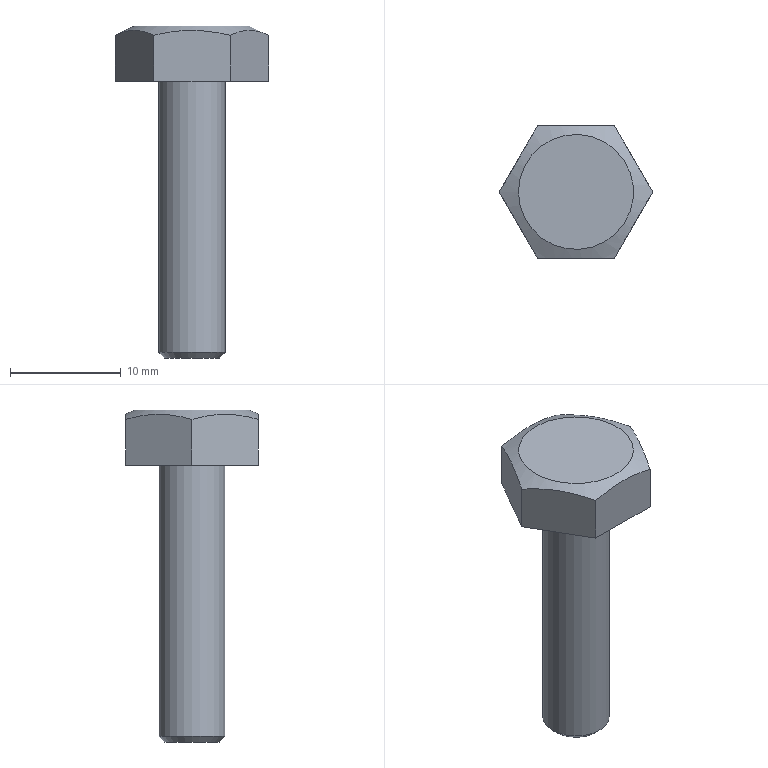Component | NX | BOLT_M6X25 | 1 solid | 12 faces | box 13.86 x 12 x 30 mm | volume 1316 mm3 | plane 9 | cone 2 | cylinder 1 | commonest cylinder face diameters 6 x1
STEP:
#1=CARTESIAN_POINT('',(0.,0.,0.));
#2=DIRECTION('',(0.,0.,1.));
#3=DIRECTION('',(1.,0.,0.));
#4=AXIS2_PLACEMENT_3D('',#1,#2,#3);
#5=CARTESIAN_POINT('',(16.5,-20.,-3.));
#6=VERTEX_POINT('',#5);
#7=CARTESIAN_POINT('',(19.,-20.,-3.));
#8=DIRECTION('',(0.,0.,-1.));
#9=DIRECTION('',(-1.,0.,0.));
#10=AXIS2_PLACEMENT_3D('',#7,#8,#9);
#11=CIRCLE('',#10,2.5);
#12=CARTESIAN_POINT('',(19.,-20.,-3.));
#13=DIRECTION('',(0.,0.,-1.));
#14=DIRECTION('',(-1.,0.,0.));
#15=AXIS2_PLACEMENT_3D('',#12,#13,#14);
#16=PLANE('',#15);
#17=CARTESIAN_POINT('',(0.,0.));
#18=DIRECTION('',(1.,0.));
#19=AXIS2_PLACEMENT_2D('',#17,#18);
#20=CIRCLE('',#19,2.5);
#21=(GEOMETRIC_REPRESENTATION_CONTEXT(2)PARAMETRIC_REPRESENTATION_CONTEXT()REPRESENTATION_CONTEXT('',''));
#22=DEFINITIONAL_REPRESENTATION('',(#20),#21);
#23=PCURVE('',#16,#22);
#24=CARTESIAN_POINT('',(19.,-20.,-2.5));
#25=DIRECTION('',(0.,0.,1.));
#26=DIRECTION('',(1.,0.,0.));
#27=AXIS2_PLACEMENT_3D('',#24,#25,#26);
#28=CONICAL_SURFACE('',#27,3.,0.7854);
#29=CARTESIAN_POINT('',(9.425,-0.5));
#30=DIRECTION('',(-1.,0.));
#31=VECTOR('',#30,1.);
#32=LINE('',#29,#31);
#33=(GEOMETRIC_REPRESENTATION_CONTEXT(2)PARAMETRIC_REPRESENTATION_CONTEXT()REPRESENTATION_CONTEXT('',''));
#34=DEFINITIONAL_REPRESENTATION('',(#32),#33);
#35=PCURVE('',#28,#34);
#36=SURFACE_CURVE('',#11,(#23,#35),.PCURVE_S1.);
#37=EDGE_CURVE('',#6,#6,#36,.T.);
#38=ORIENTED_EDGE('',*,*,#37,.T.);
#39=EDGE_LOOP('',(#38));
#40=FACE_BOUND('',#39,.T.);
#41=ADVANCED_FACE('',(#40),#16,.T.);
#42=CARTESIAN_POINT('',(16.,-20.,-2.5));
#43=VERTEX_POINT('',#42);
#44=CARTESIAN_POINT('',(22.,-20.,-2.5));
#45=VERTEX_POINT('',#44);
#46=CARTESIAN_POINT('',(19.,-20.,-2.5));
#47=DIRECTION('',(0.,0.,1.));
#48=DIRECTION('',(-1.,0.,0.));
#49=AXIS2_PLACEMENT_3D('',#46,#47,#48);
#50=CIRCLE('',#49,3.);
#51=CARTESIAN_POINT('',(19.,-20.,-3.));
#52=DIRECTION('',(0.,0.,1.));
#53=DIRECTION('',(1.,0.,0.));
#54=AXIS2_PLACEMENT_3D('',#51,#52,#53);
#55=CYLINDRICAL_SURFACE('',#54,3.);
#56=CARTESIAN_POINT('',(3.142,0.5));
#57=DIRECTION('',(1.,0.));
#58=VECTOR('',#57,1.);
#59=LINE('',#56,#58);
#60=(GEOMETRIC_REPRESENTATION_CONTEXT(2)PARAMETRIC_REPRESENTATION_CONTEXT()REPRESENTATION_CONTEXT('',''));
#61=DEFINITIONAL_REPRESENTATION('',(#59),#60);
#62=PCURVE('',#55,#61);
#63=CARTESIAN_POINT('',(3.142,0.));
#64=DIRECTION('',(1.,0.));
#65=VECTOR('',#64,1.);
#66=LINE('',#63,#65);
#67=(GEOMETRIC_REPRESENTATION_CONTEXT(2)PARAMETRIC_REPRESENTATION_CONTEXT()REPRESENTATION_CONTEXT('',''));
#68=DEFINITIONAL_REPRESENTATION('',(#66),#67);
#69=PCURVE('',#28,#68);
#70=SURFACE_CURVE('',#50,(#62,#69),.PCURVE_S1.);
#71=EDGE_CURVE('',#43,#45,#70,.T.);
#72=ORIENTED_EDGE('',*,*,#71,.T.);
#73=CARTESIAN_POINT('',(22.,-20.,22.));
#74=VERTEX_POINT('',#73);
#75=CARTESIAN_POINT('',(22.,-20.,-2.5));
#76=CARTESIAN_POINT('',(22.,-20.,22.));
#77=B_SPLINE_CURVE_WITH_KNOTS('',1,(#75,#76),.UNSPECIFIED.,.F.,.F.,(2,2),(0.5,25.),.PIECEWISE_BEZIER_KNOTS.);
#78=CARTESIAN_POINT('',(6.283,0.));
#79=DIRECTION('',(0.,1.));
#80=VECTOR('',#79,1.);
#81=LINE('',#78,#80);
#82=(GEOMETRIC_REPRESENTATION_CONTEXT(2)PARAMETRIC_REPRESENTATION_CONTEXT()REPRESENTATION_CONTEXT('',''));
#83=DEFINITIONAL_REPRESENTATION('',(#81),#82);
#84=PCURVE('',#55,#83);
#85=CARTESIAN_POINT('',(0.,0.));
#86=DIRECTION('',(0.,1.));
#87=VECTOR('',#86,1.);
#88=LINE('',#85,#87);
#89=(GEOMETRIC_REPRESENTATION_CONTEXT(2)PARAMETRIC_REPRESENTATION_CONTEXT()REPRESENTATION_CONTEXT('',''));
#90=DEFINITIONAL_REPRESENTATION('',(#88),#89);
#91=PCURVE('',#55,#90);
#92=SEAM_CURVE('',#77,(#84,#91),.PCURVE_S1.);
#93=EDGE_CURVE('',#45,#74,#92,.T.);
#94=ORIENTED_EDGE('',*,*,#93,.T.);
#95=CARTESIAN_POINT('',(19.,-20.,22.));
#96=DIRECTION('',(0.,0.,-1.));
#97=DIRECTION('',(1.,0.,0.));
#98=AXIS2_PLACEMENT_3D('',#95,#96,#97);
#99=CIRCLE('',#98,3.);
#100=CARTESIAN_POINT('',(6.283,25.));
#101=DIRECTION('',(-1.,0.));
#102=VECTOR('',#101,1.);
#103=LINE('',#100,#102);
#104=(GEOMETRIC_REPRESENTATION_CONTEXT(2)PARAMETRIC_REPRESENTATION_CONTEXT()REPRESENTATION_CONTEXT('',''));
#105=DEFINITIONAL_REPRESENTATION('',(#103),#104);
#106=PCURVE('',#55,#105);
#107=CARTESIAN_POINT('',(19.,-20.,22.));
#108=DIRECTION('',(0.,0.,1.));
#109=DIRECTION('',(1.,0.,0.));
#110=AXIS2_PLACEMENT_3D('',#107,#108,#109);
#111=PLANE('',#110);
#112=CARTESIAN_POINT('',(3.,0.));
#113=CARTESIAN_POINT('',(3.,-5.196));
#114=CARTESIAN_POINT('',(-1.5,-2.598));
#115=CARTESIAN_POINT('',(-6.,-0.));
#116=CARTESIAN_POINT('',(-1.5,2.598));
#117=CARTESIAN_POINT('',(3.,5.196));
#118=CARTESIAN_POINT('',(3.,0.));
#119=(BOUNDED_CURVE()B_SPLINE_CURVE(2,(#112,#113,#114,#115,#116,#117,#118),.UNSPECIFIED.,.T.,.F.)B_SPLINE_CURVE_WITH_KNOTS((1,2,2,2,2,1),(-2.094,0.,2.094,4.189,6.283,8.378),.UNSPECIFIED.)CURVE()GEOMETRIC_REPRESENTATION_ITEM()RATIONAL_B_SPLINE_CURVE((1.,0.5,1.,0.5,1.,0.5,1.))REPRESENTATION_ITEM(''));
#120=(GEOMETRIC_REPRESENTATION_CONTEXT(2)PARAMETRIC_REPRESENTATION_CONTEXT()REPRESENTATION_CONTEXT('',''));
#121=DEFINITIONAL_REPRESENTATION('',(#119),#120);
#122=PCURVE('',#111,#121);
#123=SURFACE_CURVE('',#99,(#106,#122),.PCURVE_S1.);
#124=EDGE_CURVE('',#74,#74,#123,.T.);
#125=ORIENTED_EDGE('',*,*,#124,.T.);
#126=ORIENTED_EDGE('',*,*,#93,.F.);
#127=CARTESIAN_POINT('',(19.,-20.,-2.5));
#128=DIRECTION('',(0.,0.,1.));
#129=DIRECTION('',(-1.,0.,0.));
#130=AXIS2_PLACEMENT_3D('',#127,#128,#129);
#131=CIRCLE('',#130,3.);
#132=CARTESIAN_POINT('',(-3.142,0.5));
#133=DIRECTION('',(1.,0.));
#134=VECTOR('',#133,1.);
#135=LINE('',#132,#134);
#136=(GEOMETRIC_REPRESENTATION_CONTEXT(2)PARAMETRIC_REPRESENTATION_CONTEXT()REPRESENTATION_CONTEXT('',''));
#137=DEFINITIONAL_REPRESENTATION('',(#135),#136);
#138=PCURVE('',#55,#137);
#139=CARTESIAN_POINT('',(3.142,0.));
#140=DIRECTION('',(1.,0.));
#141=VECTOR('',#140,1.);
#142=LINE('',#139,#141);
#143=(GEOMETRIC_REPRESENTATION_CONTEXT(2)PARAMETRIC_REPRESENTATION_CONTEXT()REPRESENTATION_CONTEXT('',''));
#144=DEFINITIONAL_REPRESENTATION('',(#142),#143);
#145=PCURVE('',#28,#144);
#146=SURFACE_CURVE('',#131,(#138,#145),.PCURVE_S1.);
#147=EDGE_CURVE('',#45,#43,#146,.T.);
#148=ORIENTED_EDGE('',*,*,#147,.T.);
#149=EDGE_LOOP('',(#72,#94,#125,#126,#148));
#150=FACE_BOUND('',#149,.T.);
#151=ADVANCED_FACE('',(#150),#55,.T.);
#152=CARTESIAN_POINT('',(15.536,-14.,26.151));
#153=VERTEX_POINT('',#152);
#154=CARTESIAN_POINT('',(15.536,-14.,22.));
#155=VERTEX_POINT('',#154);
#156=CARTESIAN_POINT('',(15.536,-14.,27.));
#157=DIRECTION('',(0.,0.,-1.));
#158=VECTOR('',#157,1.);
#159=LINE('',#156,#158);
#160=CARTESIAN_POINT('',(22.464,-14.,27.));
#161=DIRECTION('',(0.,-1.,0.));
#162=DIRECTION('',(1.,0.,0.));
#163=AXIS2_PLACEMENT_3D('',#160,#161,#162);
#164=PLANE('',#163);
#165=CARTESIAN_POINT('',(-6.928,0.));
#166=DIRECTION('',(0.,-1.));
#167=VECTOR('',#166,1.);
#168=LINE('',#165,#167);
#169=(GEOMETRIC_REPRESENTATION_CONTEXT(2)PARAMETRIC_REPRESENTATION_CONTEXT()REPRESENTATION_CONTEXT('',''));
#170=DEFINITIONAL_REPRESENTATION('',(#168),#169);
#171=PCURVE('',#164,#170);
#172=CARTESIAN_POINT('',(15.536,-14.,27.));
#173=DIRECTION('',(0.866,-0.5,0.));
#174=DIRECTION('',(0.5,0.866,0.));
#175=AXIS2_PLACEMENT_3D('',#172,#173,#174);
#176=PLANE('',#175);
#177=CARTESIAN_POINT('',(0.,0.));
#178=DIRECTION('',(0.,-1.));
#179=VECTOR('',#178,1.);
#180=LINE('',#177,#179);
#181=(GEOMETRIC_REPRESENTATION_CONTEXT(2)PARAMETRIC_REPRESENTATION_CONTEXT()REPRESENTATION_CONTEXT('',''));
#182=DEFINITIONAL_REPRESENTATION('',(#180),#181);
#183=PCURVE('',#176,#182);
#184=SURFACE_CURVE('',#159,(#171,#183),.PCURVE_S1.);
#185=EDGE_CURVE('',#153,#155,#184,.T.);
#186=ORIENTED_EDGE('',*,*,#185,.F.);
#187=CARTESIAN_POINT('',(22.464,-14.,26.151));
#188=VERTEX_POINT('',#187);
#189=CARTESIAN_POINT('',(15.536,-14.,26.151));
#190=CARTESIAN_POINT('',(16.672,-14.,26.43));
#191=CARTESIAN_POINT('',(17.839,-14.,26.606));
#192=CARTESIAN_POINT('',(20.161,-14.,26.606));
#193=CARTESIAN_POINT('',(21.337,-14.,26.427));
#194=CARTESIAN_POINT('',(22.464,-14.,26.151));
#195=B_SPLINE_CURVE_WITH_KNOTS('',3,(#189,#190,#191,#192,#193,#194),.UNSPECIFIED.,.F.,.F.,(4,2,4),(0.,0.5,1.),.UNSPECIFIED.);
#196=CARTESIAN_POINT('',(-6.928,-0.8487));
#197=CARTESIAN_POINT('',(-5.792,-0.5703));
#198=CARTESIAN_POINT('',(-4.625,-0.3939));
#199=CARTESIAN_POINT('',(-2.304,-0.3939));
#200=CARTESIAN_POINT('',(-1.127,-0.5725));
#201=CARTESIAN_POINT('',(0.,-0.8487));
#202=B_SPLINE_CURVE_WITH_KNOTS('',3,(#196,#197,#198,#199,#200,#201),.UNSPECIFIED.,.F.,.F.,(4,2,4),(0.,0.5,1.),.UNSPECIFIED.);
#203=(GEOMETRIC_REPRESENTATION_CONTEXT(2)PARAMETRIC_REPRESENTATION_CONTEXT()REPRESENTATION_CONTEXT('',''));
#204=DEFINITIONAL_REPRESENTATION('',(#202),#203);
#205=PCURVE('',#164,#204);
#206=CARTESIAN_POINT('',(19.,-20.,27.));
#207=DIRECTION('',(0.,0.,-1.));
#208=DIRECTION('',(-1.,0.,0.));
#209=AXIS2_PLACEMENT_3D('',#206,#207,#208);
#210=CONICAL_SURFACE('',#209,5.196,1.115);
#211=CARTESIAN_POINT('',(1.047,0.8487));
#212=CARTESIAN_POINT('',(1.06,0.8234));
#213=CARTESIAN_POINT('',(1.087,0.7744));
#214=CARTESIAN_POINT('',(1.128,0.7061));
#215=CARTESIAN_POINT('',(1.172,0.6434));
#216=CARTESIAN_POINT('',(1.217,0.5869));
#217=CARTESIAN_POINT('',(1.264,0.5368));
#218=CARTESIAN_POINT('',(1.313,0.4937));
#219=CARTESIAN_POINT('',(1.362,0.4578));
#220=CARTESIAN_POINT('',(1.414,0.4295));
#221=CARTESIAN_POINT('',(1.465,0.409));
#222=CARTESIAN_POINT('',(1.518,0.3967));
#223=CARTESIAN_POINT('',(1.571,0.3925));
#224=CARTESIAN_POINT('',(1.624,0.3967));
#225=CARTESIAN_POINT('',(1.676,0.4091));
#226=CARTESIAN_POINT('',(1.728,0.4296));
#227=CARTESIAN_POINT('',(1.779,0.458));
#228=CARTESIAN_POINT('',(1.829,0.4941));
#229=CARTESIAN_POINT('',(1.878,0.5374));
#230=CARTESIAN_POINT('',(1.925,0.5876));
#231=CARTESIAN_POINT('',(1.97,0.6442));
#232=CARTESIAN_POINT('',(2.014,0.7068));
#233=CARTESIAN_POINT('',(2.055,0.7749));
#234=CARTESIAN_POINT('',(2.082,0.8236));
#235=CARTESIAN_POINT('',(2.094,0.8487));
#236=B_SPLINE_CURVE_WITH_KNOTS('',3,(#211,#212,#213,#214,#215,#216,#217,#218,#219,#220,#221,#222,#223,#224,#225,#226,#227,#228,#229,#230,#231,#232,#233,#234,#235),.UNSPECIFIED.,.F.,.F.,(4,1,1,1,1,1,1,1,1,1,1,1,1,1,1,1,1,1,1,1,1,1,4),(0.,0.04545,0.09091,0.1364,0.1818,0.2273,0.2727,0.3182,0.3636,0.4091,0.4545,0.5,0.5455,0.5909,0.6364,0.6818,0.7273,0.7727,0.8182,0.8636,0.9091,0.9545,1.),.QUASI_UNIFORM_KNOTS.);
#237=(GEOMETRIC_REPRESENTATION_CONTEXT(2)PARAMETRIC_REPRESENTATION_CONTEXT()REPRESENTATION_CONTEXT('',''));
#238=DEFINITIONAL_REPRESENTATION('',(#236),#237);
#239=PCURVE('',#210,#238);
#240=SURFACE_CURVE('',#195,(#205,#239),.PCURVE_S1.);
#241=EDGE_CURVE('',#153,#188,#240,.T.);
#242=ORIENTED_EDGE('',*,*,#241,.T.);
#243=CARTESIAN_POINT('',(22.464,-14.,22.));
#244=VERTEX_POINT('',#243);
#245=CARTESIAN_POINT('',(22.464,-14.,27.));
#246=DIRECTION('',(0.,0.,-1.));
#247=VECTOR('',#246,1.);
#248=LINE('',#245,#247);
#249=CARTESIAN_POINT('',(0.,0.));
#250=DIRECTION('',(0.,-1.));
#251=VECTOR('',#250,1.);
#252=LINE('',#249,#251);
#253=(GEOMETRIC_REPRESENTATION_CONTEXT(2)PARAMETRIC_REPRESENTATION_CONTEXT()REPRESENTATION_CONTEXT('',''));
#254=DEFINITIONAL_REPRESENTATION('',(#252),#253);
#255=PCURVE('',#164,#254);
#256=CARTESIAN_POINT('',(25.928,-20.,27.));
#257=DIRECTION('',(-0.866,-0.5,0.));
#258=DIRECTION('',(0.5,-0.866,0.));
#259=AXIS2_PLACEMENT_3D('',#256,#257,#258);
#260=PLANE('',#259);
#261=CARTESIAN_POINT('',(-6.928,0.));
#262=DIRECTION('',(0.,-1.));
#263=VECTOR('',#262,1.);
#264=LINE('',#261,#263);
#265=(GEOMETRIC_REPRESENTATION_CONTEXT(2)PARAMETRIC_REPRESENTATION_CONTEXT()REPRESENTATION_CONTEXT('',''));
#266=DEFINITIONAL_REPRESENTATION('',(#264),#265);
#267=PCURVE('',#260,#266);
#268=SURFACE_CURVE('',#248,(#255,#267),.PCURVE_S1.);
#269=EDGE_CURVE('',#188,#244,#268,.T.);
#270=ORIENTED_EDGE('',*,*,#269,.T.);
#271=CARTESIAN_POINT('',(22.464,-14.,22.));
#272=DIRECTION('',(-1.,-0.,0.));
#273=VECTOR('',#272,1.);
#274=LINE('',#271,#273);
#275=CARTESIAN_POINT('',(0.,-5.));
#276=DIRECTION('',(-1.,0.));
#277=VECTOR('',#276,1.);
#278=LINE('',#275,#277);
#279=(GEOMETRIC_REPRESENTATION_CONTEXT(2)PARAMETRIC_REPRESENTATION_CONTEXT()REPRESENTATION_CONTEXT('',''));
#280=DEFINITIONAL_REPRESENTATION('',(#278),#279);
#281=PCURVE('',#164,#280);
#282=CARTESIAN_POINT('',(3.464,6.));
#283=DIRECTION('',(-1.,-0.));
#284=VECTOR('',#283,1.);
#285=LINE('',#282,#284);
#286=(GEOMETRIC_REPRESENTATION_CONTEXT(2)PARAMETRIC_REPRESENTATION_CONTEXT()REPRESENTATION_CONTEXT('',''));
#287=DEFINITIONAL_REPRESENTATION('',(#285),#286);
#288=PCURVE('',#111,#287);
#289=SURFACE_CURVE('',#274,(#281,#288),.PCURVE_S1.);
#290=EDGE_CURVE('',#244,#155,#289,.T.);
#291=ORIENTED_EDGE('',*,*,#290,.T.);
#292=EDGE_LOOP('',(#186,#242,#270,#291));
#293=FACE_BOUND('',#292,.T.);
#294=ADVANCED_FACE('',(#293),#164,.F.);
#295=CARTESIAN_POINT('',(12.072,-20.,26.151));
#296=VERTEX_POINT('',#295);
#297=CARTESIAN_POINT('',(12.072,-20.,22.));
#298=VERTEX_POINT('',#297);
#299=CARTESIAN_POINT('',(12.072,-20.,27.));
#300=DIRECTION('',(0.,0.,-1.));
#301=VECTOR('',#300,1.);
#302=LINE('',#299,#301);
#303=CARTESIAN_POINT('',(-6.928,0.));
#304=DIRECTION('',(0.,-1.));
#305=VECTOR('',#304,1.);
#306=LINE('',#303,#305);
#307=(GEOMETRIC_REPRESENTATION_CONTEXT(2)PARAMETRIC_REPRESENTATION_CONTEXT()REPRESENTATION_CONTEXT('',''));
#308=DEFINITIONAL_REPRESENTATION('',(#306),#307);
#309=PCURVE('',#176,#308);
#310=CARTESIAN_POINT('',(12.072,-20.,27.));
#311=DIRECTION('',(0.866,0.5,0.));
#312=DIRECTION('',(-0.5,0.866,0.));
#313=AXIS2_PLACEMENT_3D('',#310,#311,#312);
#314=PLANE('',#313);
#315=CARTESIAN_POINT('',(0.,0.));
#316=DIRECTION('',(0.,-1.));
#317=VECTOR('',#316,1.);
#318=LINE('',#315,#317);
#319=(GEOMETRIC_REPRESENTATION_CONTEXT(2)PARAMETRIC_REPRESENTATION_CONTEXT()REPRESENTATION_CONTEXT('',''));
#320=DEFINITIONAL_REPRESENTATION('',(#318),#319);
#321=PCURVE('',#314,#320);
#322=SURFACE_CURVE('',#302,(#309,#321),.PCURVE_S1.);
#323=EDGE_CURVE('',#296,#298,#322,.T.);
#324=ORIENTED_EDGE('',*,*,#323,.F.);
#325=CARTESIAN_POINT('',(12.072,-20.,26.151));
#326=CARTESIAN_POINT('',(12.641,-19.013,26.43));
#327=CARTESIAN_POINT('',(13.215,-18.02,26.605));
#328=CARTESIAN_POINT('',(14.376,-16.009,26.608));
#329=CARTESIAN_POINT('',(14.964,-14.99,26.431));
#330=CARTESIAN_POINT('',(15.536,-14.,26.151));
#331=B_SPLINE_CURVE_WITH_KNOTS('',3,(#325,#326,#327,#328,#329,#330),.UNSPECIFIED.,.F.,.F.,(4,2,4),(0.,0.5,1.),.UNSPECIFIED.);
#332=CARTESIAN_POINT('',(-6.928,-0.8487));
#333=CARTESIAN_POINT('',(-5.789,-0.5696));
#334=CARTESIAN_POINT('',(-4.642,-0.3955));
#335=CARTESIAN_POINT('',(-2.32,-0.3923));
#336=CARTESIAN_POINT('',(-1.144,-0.5686));
#337=CARTESIAN_POINT('',(0.,-0.8487));
#338=B_SPLINE_CURVE_WITH_KNOTS('',3,(#332,#333,#334,#335,#336,#337),.UNSPECIFIED.,.F.,.F.,(4,2,4),(0.,0.5,1.),.UNSPECIFIED.);
#339=(GEOMETRIC_REPRESENTATION_CONTEXT(2)PARAMETRIC_REPRESENTATION_CONTEXT()REPRESENTATION_CONTEXT('',''));
#340=DEFINITIONAL_REPRESENTATION('',(#338),#339);
#341=PCURVE('',#176,#340);
#342=CARTESIAN_POINT('',(0.,0.8487));
#343=CARTESIAN_POINT('',(0.01294,0.8234));
#344=CARTESIAN_POINT('',(0.03944,0.7743));
#345=CARTESIAN_POINT('',(0.08096,0.7061));
#346=CARTESIAN_POINT('',(0.1243,0.6437));
#347=CARTESIAN_POINT('',(0.1693,0.5874));
#348=CARTESIAN_POINT('',(0.2159,0.5376));
#349=CARTESIAN_POINT('',(0.2641,0.4946));
#350=CARTESIAN_POINT('',(0.3136,0.4588));
#351=CARTESIAN_POINT('',(0.3642,0.4304));
#352=CARTESIAN_POINT('',(0.4158,0.4098));
#353=CARTESIAN_POINT('',(0.4681,0.3971));
#354=CARTESIAN_POINT('',(0.5208,0.3925));
#355=CARTESIAN_POINT('',(0.5737,0.3962));
#356=CARTESIAN_POINT('',(0.6263,0.4082));
#357=CARTESIAN_POINT('',(0.6785,0.4284));
#358=CARTESIAN_POINT('',(0.7298,0.4565));
#359=CARTESIAN_POINT('',(0.78,0.4922));
#360=CARTESIAN_POINT('',(0.8289,0.5354));
#361=CARTESIAN_POINT('',(0.8762,0.5855));
#362=CARTESIAN_POINT('',(0.9218,0.6423));
#363=CARTESIAN_POINT('',(0.9657,0.7052));
#364=CARTESIAN_POINT('',(1.008,0.7739));
#365=CARTESIAN_POINT('',(1.034,0.8233));
#366=CARTESIAN_POINT('',(1.047,0.8487));
#367=B_SPLINE_CURVE_WITH_KNOTS('',3,(#342,#343,#344,#345,#346,#347,#348,#349,#350,#351,#352,#353,#354,#355,#356,#357,#358,#359,#360,#361,#362,#363,#364,#365,#366),.UNSPECIFIED.,.F.,.F.,(4,1,1,1,1,1,1,1,1,1,1,1,1,1,1,1,1,1,1,1,1,1,4),(0.,0.04545,0.09091,0.1364,0.1818,0.2273,0.2727,0.3182,0.3636,0.4091,0.4545,0.5,0.5455,0.5909,0.6364,0.6818,0.7273,0.7727,0.8182,0.8636,0.9091,0.9545,1.),.QUASI_UNIFORM_KNOTS.);
#368=(GEOMETRIC_REPRESENTATION_CONTEXT(2)PARAMETRIC_REPRESENTATION_CONTEXT()REPRESENTATION_CONTEXT('',''));
#369=DEFINITIONAL_REPRESENTATION('',(#367),#368);
#370=PCURVE('',#210,#369);
#371=SURFACE_CURVE('',#331,(#341,#370),.PCURVE_S1.);
#372=EDGE_CURVE('',#296,#153,#371,.T.);
#373=ORIENTED_EDGE('',*,*,#372,.T.);
#374=ORIENTED_EDGE('',*,*,#185,.T.);
#375=CARTESIAN_POINT('',(15.536,-14.,22.));
#376=DIRECTION('',(-0.5,-0.866,0.));
#377=VECTOR('',#376,1.);
#378=LINE('',#375,#377);
#379=CARTESIAN_POINT('',(0.,-5.));
#380=DIRECTION('',(-1.,0.));
#381=VECTOR('',#380,1.);
#382=LINE('',#379,#381);
#383=(GEOMETRIC_REPRESENTATION_CONTEXT(2)PARAMETRIC_REPRESENTATION_CONTEXT()REPRESENTATION_CONTEXT('',''));
#384=DEFINITIONAL_REPRESENTATION('',(#382),#383);
#385=PCURVE('',#176,#384);
#386=CARTESIAN_POINT('',(-3.464,6.));
#387=DIRECTION('',(-0.5,-0.866));
#388=VECTOR('',#387,1.);
#389=LINE('',#386,#388);
#390=(GEOMETRIC_REPRESENTATION_CONTEXT(2)PARAMETRIC_REPRESENTATION_CONTEXT()REPRESENTATION_CONTEXT('',''));
#391=DEFINITIONAL_REPRESENTATION('',(#389),#390);
#392=PCURVE('',#111,#391);
#393=SURFACE_CURVE('',#378,(#385,#392),.PCURVE_S1.);
#394=EDGE_CURVE('',#155,#298,#393,.T.);
#395=ORIENTED_EDGE('',*,*,#394,.T.);
#396=EDGE_LOOP('',(#324,#373,#374,#395));
#397=FACE_BOUND('',#396,.T.);
#398=ADVANCED_FACE('',(#397),#176,.F.);
#399=CARTESIAN_POINT('',(15.536,-26.,26.151));
#400=VERTEX_POINT('',#399);
#401=CARTESIAN_POINT('',(15.536,-26.,22.));
#402=VERTEX_POINT('',#401);
#403=CARTESIAN_POINT('',(15.536,-26.,27.));
#404=DIRECTION('',(0.,0.,-1.));
#405=VECTOR('',#404,1.);
#406=LINE('',#403,#405);
#407=CARTESIAN_POINT('',(-6.928,0.));
#408=DIRECTION('',(0.,-1.));
#409=VECTOR('',#408,1.);
#410=LINE('',#407,#409);
#411=(GEOMETRIC_REPRESENTATION_CONTEXT(2)PARAMETRIC_REPRESENTATION_CONTEXT()REPRESENTATION_CONTEXT('',''));
#412=DEFINITIONAL_REPRESENTATION('',(#410),#411);
#413=PCURVE('',#314,#412);
#414=CARTESIAN_POINT('',(15.536,-26.,27.));
#415=DIRECTION('',(0.,1.,0.));
#416=DIRECTION('',(-1.,0.,0.));
#417=AXIS2_PLACEMENT_3D('',#414,#415,#416);
#418=PLANE('',#417);
#419=CARTESIAN_POINT('',(0.,0.));
#420=DIRECTION('',(0.,-1.));
#421=VECTOR('',#420,1.);
#422=LINE('',#419,#421);
#423=(GEOMETRIC_REPRESENTATION_CONTEXT(2)PARAMETRIC_REPRESENTATION_CONTEXT()REPRESENTATION_CONTEXT('',''));
#424=DEFINITIONAL_REPRESENTATION('',(#422),#423);
#425=PCURVE('',#418,#424);
#426=SURFACE_CURVE('',#406,(#413,#425),.PCURVE_S1.);
#427=EDGE_CURVE('',#400,#402,#426,.T.);
#428=ORIENTED_EDGE('',*,*,#427,.F.);
#429=CARTESIAN_POINT('',(15.536,-26.,26.151));
#430=CARTESIAN_POINT('',(14.966,-25.013,26.43));
#431=CARTESIAN_POINT('',(14.393,-24.02,26.605));
#432=CARTESIAN_POINT('',(13.232,-22.009,26.608));
#433=CARTESIAN_POINT('',(12.644,-20.99,26.431));
#434=CARTESIAN_POINT('',(12.072,-20.,26.151));
#435=B_SPLINE_CURVE_WITH_KNOTS('',3,(#429,#430,#431,#432,#433,#434),.UNSPECIFIED.,.F.,.F.,(4,2,4),(0.,0.5,1.),.UNSPECIFIED.);
#436=CARTESIAN_POINT('',(-6.928,-0.8487));
#437=CARTESIAN_POINT('',(-5.789,-0.5696));
#438=CARTESIAN_POINT('',(-4.642,-0.3955));
#439=CARTESIAN_POINT('',(-2.32,-0.3923));
#440=CARTESIAN_POINT('',(-1.144,-0.5686));
#441=CARTESIAN_POINT('',(0.,-0.8487));
#442=B_SPLINE_CURVE_WITH_KNOTS('',3,(#436,#437,#438,#439,#440,#441),.UNSPECIFIED.,.F.,.F.,(4,2,4),(0.,0.5,1.),.UNSPECIFIED.);
#443=(GEOMETRIC_REPRESENTATION_CONTEXT(2)PARAMETRIC_REPRESENTATION_CONTEXT()REPRESENTATION_CONTEXT('',''));
#444=DEFINITIONAL_REPRESENTATION('',(#442),#443);
#445=PCURVE('',#314,#444);
#446=CARTESIAN_POINT('',(5.236,0.8487));
#447=CARTESIAN_POINT('',(5.249,0.8234));
#448=CARTESIAN_POINT('',(5.275,0.7743));
#449=CARTESIAN_POINT('',(5.317,0.7061));
#450=CARTESIAN_POINT('',(5.36,0.6437));
#451=CARTESIAN_POINT('',(5.405,0.5874));
#452=CARTESIAN_POINT('',(5.452,0.5376));
#453=CARTESIAN_POINT('',(5.5,0.4946));
#454=CARTESIAN_POINT('',(5.55,0.4588));
#455=CARTESIAN_POINT('',(5.6,0.4304));
#456=CARTESIAN_POINT('',(5.652,0.4098));
#457=CARTESIAN_POINT('',(5.704,0.3971));
#458=CARTESIAN_POINT('',(5.757,0.3925));
#459=CARTESIAN_POINT('',(5.81,0.3962));
#460=CARTESIAN_POINT('',(5.862,0.4082));
#461=CARTESIAN_POINT('',(5.914,0.4284));
#462=CARTESIAN_POINT('',(5.966,0.4565));
#463=CARTESIAN_POINT('',(6.016,0.4922));
#464=CARTESIAN_POINT('',(6.065,0.5354));
#465=CARTESIAN_POINT('',(6.112,0.5855));
#466=CARTESIAN_POINT('',(6.158,0.6423));
#467=CARTESIAN_POINT('',(6.202,0.7052));
#468=CARTESIAN_POINT('',(6.244,0.7739));
#469=CARTESIAN_POINT('',(6.27,0.8233));
#470=CARTESIAN_POINT('',(6.283,0.8487));
#471=B_SPLINE_CURVE_WITH_KNOTS('',3,(#446,#447,#448,#449,#450,#451,#452,#453,#454,#455,#456,#457,#458,#459,#460,#461,#462,#463,#464,#465,#466,#467,#468,#469,#470),.UNSPECIFIED.,.F.,.F.,(4,1,1,1,1,1,1,1,1,1,1,1,1,1,1,1,1,1,1,1,1,1,4),(0.,0.04545,0.09091,0.1364,0.1818,0.2273,0.2727,0.3182,0.3636,0.4091,0.4545,0.5,0.5455,0.5909,0.6364,0.6818,0.7273,0.7727,0.8182,0.8636,0.9091,0.9545,1.),.QUASI_UNIFORM_KNOTS.);
#472=(GEOMETRIC_REPRESENTATION_CONTEXT(2)PARAMETRIC_REPRESENTATION_CONTEXT()REPRESENTATION_CONTEXT('',''));
#473=DEFINITIONAL_REPRESENTATION('',(#471),#472);
#474=PCURVE('',#210,#473);
#475=SURFACE_CURVE('',#435,(#445,#474),.PCURVE_S1.);
#476=EDGE_CURVE('',#400,#296,#475,.T.);
#477=ORIENTED_EDGE('',*,*,#476,.T.);
#478=ORIENTED_EDGE('',*,*,#323,.T.);
#479=CARTESIAN_POINT('',(12.072,-20.,22.));
#480=DIRECTION('',(0.5,-0.866,0.));
#481=VECTOR('',#480,1.);
#482=LINE('',#479,#481);
#483=CARTESIAN_POINT('',(0.,-5.));
#484=DIRECTION('',(-1.,0.));
#485=VECTOR('',#484,1.);
#486=LINE('',#483,#485);
#487=(GEOMETRIC_REPRESENTATION_CONTEXT(2)PARAMETRIC_REPRESENTATION_CONTEXT()REPRESENTATION_CONTEXT('',''));
#488=DEFINITIONAL_REPRESENTATION('',(#486),#487);
#489=PCURVE('',#314,#488);
#490=CARTESIAN_POINT('',(-6.928,0.));
#491=DIRECTION('',(0.5,-0.866));
#492=VECTOR('',#491,1.);
#493=LINE('',#490,#492);
#494=(GEOMETRIC_REPRESENTATION_CONTEXT(2)PARAMETRIC_REPRESENTATION_CONTEXT()REPRESENTATION_CONTEXT('',''));
#495=DEFINITIONAL_REPRESENTATION('',(#493),#494);
#496=PCURVE('',#111,#495);
#497=SURFACE_CURVE('',#482,(#489,#496),.PCURVE_S1.);
#498=EDGE_CURVE('',#298,#402,#497,.T.);
#499=ORIENTED_EDGE('',*,*,#498,.T.);
#500=EDGE_LOOP('',(#428,#477,#478,#499));
#501=FACE_BOUND('',#500,.T.);
#502=ADVANCED_FACE('',(#501),#314,.F.);
#503=CARTESIAN_POINT('',(22.464,-26.,26.151));
#504=VERTEX_POINT('',#503);
#505=CARTESIAN_POINT('',(22.464,-26.,22.));
#506=VERTEX_POINT('',#505);
#507=CARTESIAN_POINT('',(22.464,-26.,27.));
#508=DIRECTION('',(0.,0.,-1.));
#509=VECTOR('',#508,1.);
#510=LINE('',#507,#509);
#511=CARTESIAN_POINT('',(-6.928,0.));
#512=DIRECTION('',(0.,-1.));
#513=VECTOR('',#512,1.);
#514=LINE('',#511,#513);
#515=(GEOMETRIC_REPRESENTATION_CONTEXT(2)PARAMETRIC_REPRESENTATION_CONTEXT()REPRESENTATION_CONTEXT('',''));
#516=DEFINITIONAL_REPRESENTATION('',(#514),#515);
#517=PCURVE('',#418,#516);
#518=CARTESIAN_POINT('',(22.464,-26.,27.));
#519=DIRECTION('',(-0.866,0.5,0.));
#520=DIRECTION('',(-0.5,-0.866,0.));
#521=AXIS2_PLACEMENT_3D('',#518,#519,#520);
#522=PLANE('',#521);
#523=CARTESIAN_POINT('',(0.,0.));
#524=DIRECTION('',(0.,-1.));
#525=VECTOR('',#524,1.);
#526=LINE('',#523,#525);
#527=(GEOMETRIC_REPRESENTATION_CONTEXT(2)PARAMETRIC_REPRESENTATION_CONTEXT()REPRESENTATION_CONTEXT('',''));
#528=DEFINITIONAL_REPRESENTATION('',(#526),#527);
#529=PCURVE('',#522,#528);
#530=SURFACE_CURVE('',#510,(#517,#529),.PCURVE_S1.);
#531=EDGE_CURVE('',#504,#506,#530,.T.);
#532=ORIENTED_EDGE('',*,*,#531,.F.);
#533=CARTESIAN_POINT('',(22.464,-26.,26.151));
#534=CARTESIAN_POINT('',(21.337,-26.,26.427));
#535=CARTESIAN_POINT('',(20.161,-26.,26.606));
#536=CARTESIAN_POINT('',(17.839,-26.,26.606));
#537=CARTESIAN_POINT('',(16.672,-26.,26.43));
#538=CARTESIAN_POINT('',(15.536,-26.,26.151));
#539=B_SPLINE_CURVE_WITH_KNOTS('',3,(#533,#534,#535,#536,#537,#538),.UNSPECIFIED.,.F.,.F.,(4,2,4),(0.,0.5,1.),.UNSPECIFIED.);
#540=CARTESIAN_POINT('',(-6.928,-0.8487));
#541=CARTESIAN_POINT('',(-5.801,-0.5725));
#542=CARTESIAN_POINT('',(-4.625,-0.3939));
#543=CARTESIAN_POINT('',(-2.303,-0.3939));
#544=CARTESIAN_POINT('',(-1.137,-0.5703));
#545=CARTESIAN_POINT('',(0.,-0.8487));
#546=B_SPLINE_CURVE_WITH_KNOTS('',3,(#540,#541,#542,#543,#544,#545),.UNSPECIFIED.,.F.,.F.,(4,2,4),(0.,0.5,1.),.UNSPECIFIED.);
#547=(GEOMETRIC_REPRESENTATION_CONTEXT(2)PARAMETRIC_REPRESENTATION_CONTEXT()REPRESENTATION_CONTEXT('',''));
#548=DEFINITIONAL_REPRESENTATION('',(#546),#547);
#549=PCURVE('',#418,#548);
#550=CARTESIAN_POINT('',(4.189,0.8487));
#551=CARTESIAN_POINT('',(4.202,0.8236));
#552=CARTESIAN_POINT('',(4.228,0.7749));
#553=CARTESIAN_POINT('',(4.269,0.7068));
#554=CARTESIAN_POINT('',(4.313,0.6442));
#555=CARTESIAN_POINT('',(4.358,0.5876));
#556=CARTESIAN_POINT('',(4.405,0.5374));
#557=CARTESIAN_POINT('',(4.454,0.4941));
#558=CARTESIAN_POINT('',(4.504,0.458));
#559=CARTESIAN_POINT('',(4.555,0.4296));
#560=CARTESIAN_POINT('',(4.607,0.4091));
#561=CARTESIAN_POINT('',(4.66,0.3967));
#562=CARTESIAN_POINT('',(4.712,0.3925));
#563=CARTESIAN_POINT('',(4.765,0.3967));
#564=CARTESIAN_POINT('',(4.818,0.409));
#565=CARTESIAN_POINT('',(4.87,0.4295));
#566=CARTESIAN_POINT('',(4.921,0.4578));
#567=CARTESIAN_POINT('',(4.971,0.4937));
#568=CARTESIAN_POINT('',(5.019,0.5368));
#569=CARTESIAN_POINT('',(5.066,0.5869));
#570=CARTESIAN_POINT('',(5.111,0.6434));
#571=CARTESIAN_POINT('',(5.155,0.7061));
#572=CARTESIAN_POINT('',(5.197,0.7744));
#573=CARTESIAN_POINT('',(5.223,0.8234));
#574=CARTESIAN_POINT('',(5.236,0.8487));
#575=B_SPLINE_CURVE_WITH_KNOTS('',3,(#550,#551,#552,#553,#554,#555,#556,#557,#558,#559,#560,#561,#562,#563,#564,#565,#566,#567,#568,#569,#570,#571,#572,#573,#574),.UNSPECIFIED.,.F.,.F.,(4,1,1,1,1,1,1,1,1,1,1,1,1,1,1,1,1,1,1,1,1,1,4),(0.,0.04545,0.09091,0.1364,0.1818,0.2273,0.2727,0.3182,0.3636,0.4091,0.4545,0.5,0.5455,0.5909,0.6364,0.6818,0.7273,0.7727,0.8182,0.8636,0.9091,0.9545,1.),.QUASI_UNIFORM_KNOTS.);
#576=(GEOMETRIC_REPRESENTATION_CONTEXT(2)PARAMETRIC_REPRESENTATION_CONTEXT()REPRESENTATION_CONTEXT('',''));
#577=DEFINITIONAL_REPRESENTATION('',(#575),#576);
#578=PCURVE('',#210,#577);
#579=SURFACE_CURVE('',#539,(#549,#578),.PCURVE_S1.);
#580=EDGE_CURVE('',#504,#400,#579,.T.);
#581=ORIENTED_EDGE('',*,*,#580,.T.);
#582=ORIENTED_EDGE('',*,*,#427,.T.);
#583=CARTESIAN_POINT('',(15.536,-26.,22.));
#584=DIRECTION('',(1.,-0.,0.));
#585=VECTOR('',#584,1.);
#586=LINE('',#583,#585);
#587=CARTESIAN_POINT('',(0.,-5.));
#588=DIRECTION('',(-1.,0.));
#589=VECTOR('',#588,1.);
#590=LINE('',#587,#589);
#591=(GEOMETRIC_REPRESENTATION_CONTEXT(2)PARAMETRIC_REPRESENTATION_CONTEXT()REPRESENTATION_CONTEXT('',''));
#592=DEFINITIONAL_REPRESENTATION('',(#590),#591);
#593=PCURVE('',#418,#592);
#594=CARTESIAN_POINT('',(-3.464,-6.));
#595=DIRECTION('',(1.,-0.));
#596=VECTOR('',#595,1.);
#597=LINE('',#594,#596);
#598=(GEOMETRIC_REPRESENTATION_CONTEXT(2)PARAMETRIC_REPRESENTATION_CONTEXT()REPRESENTATION_CONTEXT('',''));
#599=DEFINITIONAL_REPRESENTATION('',(#597),#598);
#600=PCURVE('',#111,#599);
#601=SURFACE_CURVE('',#586,(#593,#600),.PCURVE_S1.);
#602=EDGE_CURVE('',#402,#506,#601,.T.);
#603=ORIENTED_EDGE('',*,*,#602,.T.);
#604=EDGE_LOOP('',(#532,#581,#582,#603));
#605=FACE_BOUND('',#604,.T.);
#606=ADVANCED_FACE('',(#605),#418,.F.);
#607=CARTESIAN_POINT('',(25.928,-20.,26.151));
#608=VERTEX_POINT('',#607);
#609=CARTESIAN_POINT('',(25.928,-20.,22.));
#610=VERTEX_POINT('',#609);
#611=CARTESIAN_POINT('',(25.928,-20.,27.));
#612=DIRECTION('',(0.,0.,-1.));
#613=VECTOR('',#612,1.);
#614=LINE('',#611,#613);
#615=CARTESIAN_POINT('',(-6.928,0.));
#616=DIRECTION('',(0.,-1.));
#617=VECTOR('',#616,1.);
#618=LINE('',#615,#617);
#619=(GEOMETRIC_REPRESENTATION_CONTEXT(2)PARAMETRIC_REPRESENTATION_CONTEXT()REPRESENTATION_CONTEXT('',''));
#620=DEFINITIONAL_REPRESENTATION('',(#618),#619);
#621=PCURVE('',#522,#620);
#622=CARTESIAN_POINT('',(0.,0.));
#623=DIRECTION('',(0.,-1.));
#624=VECTOR('',#623,1.);
#625=LINE('',#622,#624);
#626=(GEOMETRIC_REPRESENTATION_CONTEXT(2)PARAMETRIC_REPRESENTATION_CONTEXT()REPRESENTATION_CONTEXT('',''));
#627=DEFINITIONAL_REPRESENTATION('',(#625),#626);
#628=PCURVE('',#260,#627);
#629=SURFACE_CURVE('',#614,(#621,#628),.PCURVE_S1.);
#630=EDGE_CURVE('',#608,#610,#629,.T.);
#631=ORIENTED_EDGE('',*,*,#630,.F.);
#632=CARTESIAN_POINT('',(25.928,-20.,26.151));
#633=CARTESIAN_POINT('',(25.359,-20.987,26.43));
#634=CARTESIAN_POINT('',(24.785,-21.98,26.605));
#635=CARTESIAN_POINT('',(23.624,-23.991,26.608));
#636=CARTESIAN_POINT('',(23.036,-25.01,26.431));
#637=CARTESIAN_POINT('',(22.464,-26.,26.151));
#638=B_SPLINE_CURVE_WITH_KNOTS('',3,(#632,#633,#634,#635,#636,#637),.UNSPECIFIED.,.F.,.F.,(4,2,4),(0.,0.5,1.),.UNSPECIFIED.);
#639=CARTESIAN_POINT('',(-6.928,-0.8487));
#640=CARTESIAN_POINT('',(-5.789,-0.5696));
#641=CARTESIAN_POINT('',(-4.642,-0.3955));
#642=CARTESIAN_POINT('',(-2.32,-0.3923));
#643=CARTESIAN_POINT('',(-1.144,-0.5686));
#644=CARTESIAN_POINT('',(0.,-0.8487));
#645=B_SPLINE_CURVE_WITH_KNOTS('',3,(#639,#640,#641,#642,#643,#644),.UNSPECIFIED.,.F.,.F.,(4,2,4),(0.,0.5,1.),.UNSPECIFIED.);
#646=(GEOMETRIC_REPRESENTATION_CONTEXT(2)PARAMETRIC_REPRESENTATION_CONTEXT()REPRESENTATION_CONTEXT('',''));
#647=DEFINITIONAL_REPRESENTATION('',(#645),#646);
#648=PCURVE('',#522,#647);
#649=CARTESIAN_POINT('',(3.142,0.8487));
#650=CARTESIAN_POINT('',(3.155,0.8234));
#651=CARTESIAN_POINT('',(3.181,0.7743));
#652=CARTESIAN_POINT('',(3.223,0.7061));
#653=CARTESIAN_POINT('',(3.266,0.6437));
#654=CARTESIAN_POINT('',(3.311,0.5874));
#655=CARTESIAN_POINT('',(3.357,0.5376));
#656=CARTESIAN_POINT('',(3.406,0.4946));
#657=CARTESIAN_POINT('',(3.455,0.4588));
#658=CARTESIAN_POINT('',(3.506,0.4304));
#659=CARTESIAN_POINT('',(3.557,0.4098));
#660=CARTESIAN_POINT('',(3.61,0.3971));
#661=CARTESIAN_POINT('',(3.662,0.3925));
#662=CARTESIAN_POINT('',(3.715,0.3962));
#663=CARTESIAN_POINT('',(3.768,0.4082));
#664=CARTESIAN_POINT('',(3.82,0.4284));
#665=CARTESIAN_POINT('',(3.871,0.4565));
#666=CARTESIAN_POINT('',(3.922,0.4922));
#667=CARTESIAN_POINT('',(3.97,0.5354));
#668=CARTESIAN_POINT('',(4.018,0.5855));
#669=CARTESIAN_POINT('',(4.063,0.6423));
#670=CARTESIAN_POINT('',(4.107,0.7052));
#671=CARTESIAN_POINT('',(4.149,0.7739));
#672=CARTESIAN_POINT('',(4.176,0.8233));
#673=CARTESIAN_POINT('',(4.189,0.8487));
#674=B_SPLINE_CURVE_WITH_KNOTS('',3,(#649,#650,#651,#652,#653,#654,#655,#656,#657,#658,#659,#660,#661,#662,#663,#664,#665,#666,#667,#668,#669,#670,#671,#672,#673),.UNSPECIFIED.,.F.,.F.,(4,1,1,1,1,1,1,1,1,1,1,1,1,1,1,1,1,1,1,1,1,1,4),(0.,0.04545,0.09091,0.1364,0.1818,0.2273,0.2727,0.3182,0.3636,0.4091,0.4545,0.5,0.5455,0.5909,0.6364,0.6818,0.7273,0.7727,0.8182,0.8636,0.9091,0.9545,1.),.QUASI_UNIFORM_KNOTS.);
#675=(GEOMETRIC_REPRESENTATION_CONTEXT(2)PARAMETRIC_REPRESENTATION_CONTEXT()REPRESENTATION_CONTEXT('',''));
#676=DEFINITIONAL_REPRESENTATION('',(#674),#675);
#677=PCURVE('',#210,#676);
#678=SURFACE_CURVE('',#638,(#648,#677),.PCURVE_S1.);
#679=EDGE_CURVE('',#608,#504,#678,.T.);
#680=ORIENTED_EDGE('',*,*,#679,.T.);
#681=ORIENTED_EDGE('',*,*,#531,.T.);
#682=CARTESIAN_POINT('',(22.464,-26.,22.));
#683=DIRECTION('',(0.5,0.866,0.));
#684=VECTOR('',#683,1.);
#685=LINE('',#682,#684);
#686=CARTESIAN_POINT('',(0.,-5.));
#687=DIRECTION('',(-1.,0.));
#688=VECTOR('',#687,1.);
#689=LINE('',#686,#688);
#690=(GEOMETRIC_REPRESENTATION_CONTEXT(2)PARAMETRIC_REPRESENTATION_CONTEXT()REPRESENTATION_CONTEXT('',''));
#691=DEFINITIONAL_REPRESENTATION('',(#689),#690);
#692=PCURVE('',#522,#691);
#693=CARTESIAN_POINT('',(3.464,-6.));
#694=DIRECTION('',(0.5,0.866));
#695=VECTOR('',#694,1.);
#696=LINE('',#693,#695);
#697=(GEOMETRIC_REPRESENTATION_CONTEXT(2)PARAMETRIC_REPRESENTATION_CONTEXT()REPRESENTATION_CONTEXT('',''));
#698=DEFINITIONAL_REPRESENTATION('',(#696),#697);
#699=PCURVE('',#111,#698);
#700=SURFACE_CURVE('',#685,(#692,#699),.PCURVE_S1.);
#701=EDGE_CURVE('',#506,#610,#700,.T.);
#702=ORIENTED_EDGE('',*,*,#701,.T.);
#703=EDGE_LOOP('',(#631,#680,#681,#702));
#704=FACE_BOUND('',#703,.T.);
#705=ADVANCED_FACE('',(#704),#522,.F.);
#706=ORIENTED_EDGE('',*,*,#269,.F.);
#707=CARTESIAN_POINT('',(22.464,-14.,26.151));
#708=CARTESIAN_POINT('',(23.034,-14.987,26.43));
#709=CARTESIAN_POINT('',(23.607,-15.98,26.605));
#710=CARTESIAN_POINT('',(24.768,-17.991,26.608));
#711=CARTESIAN_POINT('',(25.356,-19.01,26.431));
#712=CARTESIAN_POINT('',(25.928,-20.,26.151));
#713=B_SPLINE_CURVE_WITH_KNOTS('',3,(#707,#708,#709,#710,#711,#712),.UNSPECIFIED.,.F.,.F.,(4,2,4),(0.,0.5,1.),.UNSPECIFIED.);
#714=CARTESIAN_POINT('',(-6.928,-0.8487));
#715=CARTESIAN_POINT('',(-5.789,-0.5696));
#716=CARTESIAN_POINT('',(-4.642,-0.3955));
#717=CARTESIAN_POINT('',(-2.32,-0.3923));
#718=CARTESIAN_POINT('',(-1.144,-0.5686));
#719=CARTESIAN_POINT('',(0.,-0.8487));
#720=B_SPLINE_CURVE_WITH_KNOTS('',3,(#714,#715,#716,#717,#718,#719),.UNSPECIFIED.,.F.,.F.,(4,2,4),(0.,0.5,1.),.UNSPECIFIED.);
#721=(GEOMETRIC_REPRESENTATION_CONTEXT(2)PARAMETRIC_REPRESENTATION_CONTEXT()REPRESENTATION_CONTEXT('',''));
#722=DEFINITIONAL_REPRESENTATION('',(#720),#721);
#723=PCURVE('',#260,#722);
#724=CARTESIAN_POINT('',(2.094,0.8487));
#725=CARTESIAN_POINT('',(2.107,0.8234));
#726=CARTESIAN_POINT('',(2.134,0.7743));
#727=CARTESIAN_POINT('',(2.175,0.7061));
#728=CARTESIAN_POINT('',(2.219,0.6437));
#729=CARTESIAN_POINT('',(2.264,0.5874));
#730=CARTESIAN_POINT('',(2.31,0.5376));
#731=CARTESIAN_POINT('',(2.358,0.4946));
#732=CARTESIAN_POINT('',(2.408,0.4588));
#733=CARTESIAN_POINT('',(2.459,0.4304));
#734=CARTESIAN_POINT('',(2.51,0.4098));
#735=CARTESIAN_POINT('',(2.563,0.3971));
#736=CARTESIAN_POINT('',(2.615,0.3925));
#737=CARTESIAN_POINT('',(2.668,0.3962));
#738=CARTESIAN_POINT('',(2.721,0.4082));
#739=CARTESIAN_POINT('',(2.773,0.4284));
#740=CARTESIAN_POINT('',(2.824,0.4565));
#741=CARTESIAN_POINT('',(2.874,0.4922));
#742=CARTESIAN_POINT('',(2.923,0.5354));
#743=CARTESIAN_POINT('',(2.971,0.5855));
#744=CARTESIAN_POINT('',(3.016,0.6423));
#745=CARTESIAN_POINT('',(3.06,0.7052));
#746=CARTESIAN_POINT('',(3.102,0.7739));
#747=CARTESIAN_POINT('',(3.129,0.8233));
#748=CARTESIAN_POINT('',(3.142,0.8487));
#749=B_SPLINE_CURVE_WITH_KNOTS('',3,(#724,#725,#726,#727,#728,#729,#730,#731,#732,#733,#734,#735,#736,#737,#738,#739,#740,#741,#742,#743,#744,#745,#746,#747,#748),.UNSPECIFIED.,.F.,.F.,(4,1,1,1,1,1,1,1,1,1,1,1,1,1,1,1,1,1,1,1,1,1,4),(0.,0.04545,0.09091,0.1364,0.1818,0.2273,0.2727,0.3182,0.3636,0.4091,0.4545,0.5,0.5455,0.5909,0.6364,0.6818,0.7273,0.7727,0.8182,0.8636,0.9091,0.9545,1.),.QUASI_UNIFORM_KNOTS.);
#750=(GEOMETRIC_REPRESENTATION_CONTEXT(2)PARAMETRIC_REPRESENTATION_CONTEXT()REPRESENTATION_CONTEXT('',''));
#751=DEFINITIONAL_REPRESENTATION('',(#749),#750);
#752=PCURVE('',#210,#751);
#753=SURFACE_CURVE('',#713,(#723,#752),.PCURVE_S1.);
#754=EDGE_CURVE('',#188,#608,#753,.T.);
#755=ORIENTED_EDGE('',*,*,#754,.T.);
#756=ORIENTED_EDGE('',*,*,#630,.T.);
#757=CARTESIAN_POINT('',(25.928,-20.,22.));
#758=DIRECTION('',(-0.5,0.866,0.));
#759=VECTOR('',#758,1.);
#760=LINE('',#757,#759);
#761=CARTESIAN_POINT('',(0.,-5.));
#762=DIRECTION('',(-1.,0.));
#763=VECTOR('',#762,1.);
#764=LINE('',#761,#763);
#765=(GEOMETRIC_REPRESENTATION_CONTEXT(2)PARAMETRIC_REPRESENTATION_CONTEXT()REPRESENTATION_CONTEXT('',''));
#766=DEFINITIONAL_REPRESENTATION('',(#764),#765);
#767=PCURVE('',#260,#766);
#768=CARTESIAN_POINT('',(6.928,0.));
#769=DIRECTION('',(-0.5,0.866));
#770=VECTOR('',#769,1.);
#771=LINE('',#768,#770);
#772=(GEOMETRIC_REPRESENTATION_CONTEXT(2)PARAMETRIC_REPRESENTATION_CONTEXT()REPRESENTATION_CONTEXT('',''));
#773=DEFINITIONAL_REPRESENTATION('',(#771),#772);
#774=PCURVE('',#111,#773);
#775=SURFACE_CURVE('',#760,(#767,#774),.PCURVE_S1.);
#776=EDGE_CURVE('',#610,#244,#775,.T.);
#777=ORIENTED_EDGE('',*,*,#776,.T.);
#778=EDGE_LOOP('',(#706,#755,#756,#777));
#779=FACE_BOUND('',#778,.T.);
#780=ADVANCED_FACE('',(#779),#260,.F.);
#781=ORIENTED_EDGE('',*,*,#124,.F.);
#782=EDGE_LOOP('',(#781));
#783=FACE_BOUND('',#782,.T.);
#784=ORIENTED_EDGE('',*,*,#290,.F.);
#785=ORIENTED_EDGE('',*,*,#776,.F.);
#786=ORIENTED_EDGE('',*,*,#701,.F.);
#787=ORIENTED_EDGE('',*,*,#602,.F.);
#788=ORIENTED_EDGE('',*,*,#498,.F.);
#789=ORIENTED_EDGE('',*,*,#394,.F.);
#790=EDGE_LOOP('',(#784,#785,#786,#787,#788,#789));
#791=FACE_BOUND('',#790,.T.);
#792=ADVANCED_FACE('',(#783,#791),#111,.F.);
#793=ORIENTED_EDGE('',*,*,#37,.F.);
#794=CARTESIAN_POINT('',(16.5,-20.,-3.));
#795=CARTESIAN_POINT('',(16.,-20.,-2.5));
#796=B_SPLINE_CURVE_WITH_KNOTS('',1,(#794,#795),.UNSPECIFIED.,.F.,.F.,(2,2),(-0.7071,0.),.PIECEWISE_BEZIER_KNOTS.);
#797=CARTESIAN_POINT('',(9.425,0.));
#798=DIRECTION('',(0.,1.));
#799=VECTOR('',#798,1.);
#800=LINE('',#797,#799);
#801=(GEOMETRIC_REPRESENTATION_CONTEXT(2)PARAMETRIC_REPRESENTATION_CONTEXT()REPRESENTATION_CONTEXT('',''));
#802=DEFINITIONAL_REPRESENTATION('',(#800),#801);
#803=PCURVE('',#28,#802);
#804=CARTESIAN_POINT('',(3.142,0.));
#805=DIRECTION('',(0.,1.));
#806=VECTOR('',#805,1.);
#807=LINE('',#804,#806);
#808=(GEOMETRIC_REPRESENTATION_CONTEXT(2)PARAMETRIC_REPRESENTATION_CONTEXT()REPRESENTATION_CONTEXT('',''));
#809=DEFINITIONAL_REPRESENTATION('',(#807),#808);
#810=PCURVE('',#28,#809);
#811=SEAM_CURVE('',#796,(#803,#810),.PCURVE_S1.);
#812=EDGE_CURVE('',#6,#43,#811,.T.);
#813=ORIENTED_EDGE('',*,*,#812,.T.);
#814=ORIENTED_EDGE('',*,*,#147,.F.);
#815=ORIENTED_EDGE('',*,*,#71,.F.);
#816=ORIENTED_EDGE('',*,*,#812,.F.);
#817=EDGE_LOOP('',(#793,#813,#814,#815,#816));
#818=FACE_BOUND('',#817,.T.);
#819=ADVANCED_FACE('',(#818),#28,.T.);
#820=CARTESIAN_POINT('',(13.804,-20.,27.));
#821=VERTEX_POINT('',#820);
#822=CARTESIAN_POINT('',(19.,-20.,27.));
#823=DIRECTION('',(0.,0.,-1.));
#824=DIRECTION('',(-1.,0.,0.));
#825=AXIS2_PLACEMENT_3D('',#822,#823,#824);
#826=CIRCLE('',#825,5.196);
#827=CARTESIAN_POINT('',(0.,0.));
#828=DIRECTION('',(1.,0.));
#829=VECTOR('',#828,1.);
#830=LINE('',#827,#829);
#831=(GEOMETRIC_REPRESENTATION_CONTEXT(2)PARAMETRIC_REPRESENTATION_CONTEXT()REPRESENTATION_CONTEXT('',''));
#832=DEFINITIONAL_REPRESENTATION('',(#830),#831);
#833=PCURVE('',#210,#832);
#834=CARTESIAN_POINT('',(19.,-20.,27.));
#835=DIRECTION('',(0.,0.,1.));
#836=DIRECTION('',(1.,0.,0.));
#837=AXIS2_PLACEMENT_3D('',#834,#835,#836);
#838=PLANE('',#837);
#839=CARTESIAN_POINT('',(-5.196,0.));
#840=CARTESIAN_POINT('',(-5.196,9.));
#841=CARTESIAN_POINT('',(2.598,4.5));
#842=CARTESIAN_POINT('',(10.392,0.));
#843=CARTESIAN_POINT('',(2.598,-4.5));
#844=CARTESIAN_POINT('',(-5.196,-9.));
#845=CARTESIAN_POINT('',(-5.196,0.));
#846=(BOUNDED_CURVE()B_SPLINE_CURVE(2,(#839,#840,#841,#842,#843,#844,#845),.UNSPECIFIED.,.T.,.F.)B_SPLINE_CURVE_WITH_KNOTS((1,2,2,2,2,1),(-2.094,0.,2.094,4.189,6.283,8.378),.UNSPECIFIED.)CURVE()GEOMETRIC_REPRESENTATION_ITEM()RATIONAL_B_SPLINE_CURVE((1.,0.5,1.,0.5,1.,0.5,1.))REPRESENTATION_ITEM(''));
#847=(GEOMETRIC_REPRESENTATION_CONTEXT(2)PARAMETRIC_REPRESENTATION_CONTEXT()REPRESENTATION_CONTEXT('',''));
#848=DEFINITIONAL_REPRESENTATION('',(#846),#847);
#849=PCURVE('',#838,#848);
#850=SURFACE_CURVE('',#826,(#833,#849),.PCURVE_S1.);
#851=EDGE_CURVE('',#821,#821,#850,.T.);
#852=ORIENTED_EDGE('',*,*,#851,.T.);
#853=CARTESIAN_POINT('',(13.804,-20.,27.));
#854=CARTESIAN_POINT('',(12.072,-20.,26.151));
#855=B_SPLINE_CURVE_WITH_KNOTS('',1,(#853,#854),.UNSPECIFIED.,.F.,.F.,(2,2),(0.,1.929),.PIECEWISE_BEZIER_KNOTS.);
#856=CARTESIAN_POINT('',(6.283,0.));
#857=DIRECTION('',(0.,1.));
#858=VECTOR('',#857,1.);
#859=LINE('',#856,#858);
#860=(GEOMETRIC_REPRESENTATION_CONTEXT(2)PARAMETRIC_REPRESENTATION_CONTEXT()REPRESENTATION_CONTEXT('',''));
#861=DEFINITIONAL_REPRESENTATION('',(#859),#860);
#862=PCURVE('',#210,#861);
#863=CARTESIAN_POINT('',(0.,0.));
#864=DIRECTION('',(0.,1.));
#865=VECTOR('',#864,1.);
#866=LINE('',#863,#865);
#867=(GEOMETRIC_REPRESENTATION_CONTEXT(2)PARAMETRIC_REPRESENTATION_CONTEXT()REPRESENTATION_CONTEXT('',''));
#868=DEFINITIONAL_REPRESENTATION('',(#866),#867);
#869=PCURVE('',#210,#868);
#870=SEAM_CURVE('',#855,(#862,#869),.PCURVE_S1.);
#871=EDGE_CURVE('',#821,#296,#870,.T.);
#872=ORIENTED_EDGE('',*,*,#871,.T.);
#873=ORIENTED_EDGE('',*,*,#476,.F.);
#874=ORIENTED_EDGE('',*,*,#580,.F.);
#875=ORIENTED_EDGE('',*,*,#679,.F.);
#876=ORIENTED_EDGE('',*,*,#754,.F.);
#877=ORIENTED_EDGE('',*,*,#241,.F.);
#878=ORIENTED_EDGE('',*,*,#372,.F.);
#879=ORIENTED_EDGE('',*,*,#871,.F.);
#880=EDGE_LOOP('',(#852,#872,#873,#874,#875,#876,#877,#878,#879));
#881=FACE_BOUND('',#880,.T.);
#882=ADVANCED_FACE('',(#881),#210,.T.);
#883=ORIENTED_EDGE('',*,*,#851,.F.);
#884=EDGE_LOOP('',(#883));
#885=FACE_BOUND('',#884,.T.);
#886=ADVANCED_FACE('',(#885),#838,.T.);
#887=CLOSED_SHELL('',(#41,#151,#294,#398,#502,#606,#705,#780,#792,#819,#882,#886));
#888=MANIFOLD_SOLID_BREP('',#887);
#889=(LENGTH_UNIT()NAMED_UNIT(*)SI_UNIT(.MILLI.,.METRE.));
#890=UNCERTAINTY_MEASURE_WITH_UNIT(LENGTH_MEASURE(0.0005),#889,'','');
#891=(NAMED_UNIT(*)PLANE_ANGLE_UNIT()SI_UNIT($,.RADIAN.));
#892=(NAMED_UNIT(*)SI_UNIT($,.STERADIAN.)SOLID_ANGLE_UNIT());
#893=(GEOMETRIC_REPRESENTATION_CONTEXT(3)GLOBAL_UNCERTAINTY_ASSIGNED_CONTEXT((#890))GLOBAL_UNIT_ASSIGNED_CONTEXT((#889,#891,#892))REPRESENTATION_CONTEXT('',''));
#894=ADVANCED_BREP_SHAPE_REPRESENTATION('',(#4,#888),#893);